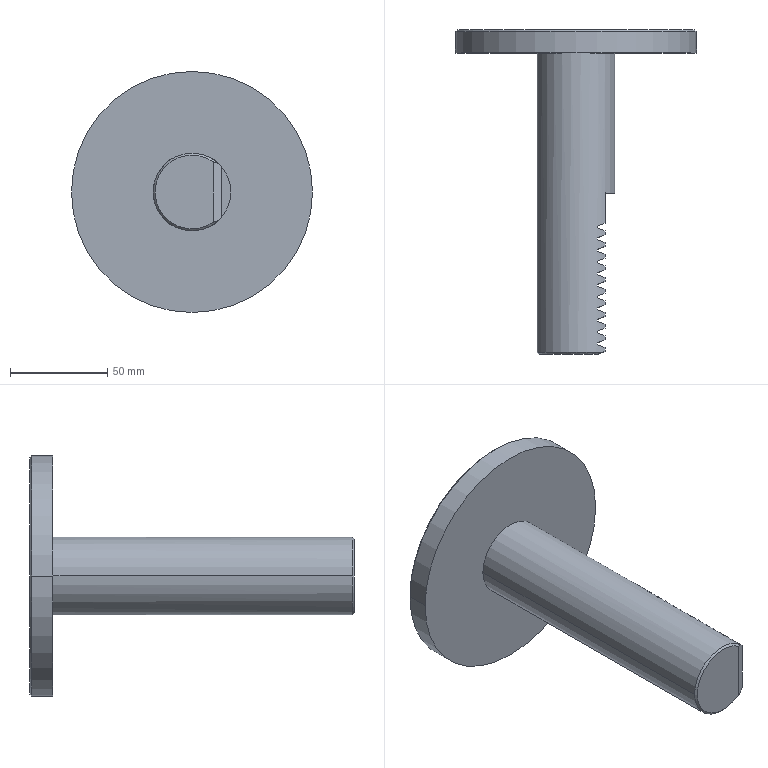Component | SolidWorks | LocatingAxis-2 | 1 solid | 64 faces | volume 318870 mm3 | plane 51 | cylinder 8 | cone 5 | commonest cylinder face diameters 40 x4 124 x2 14 x2